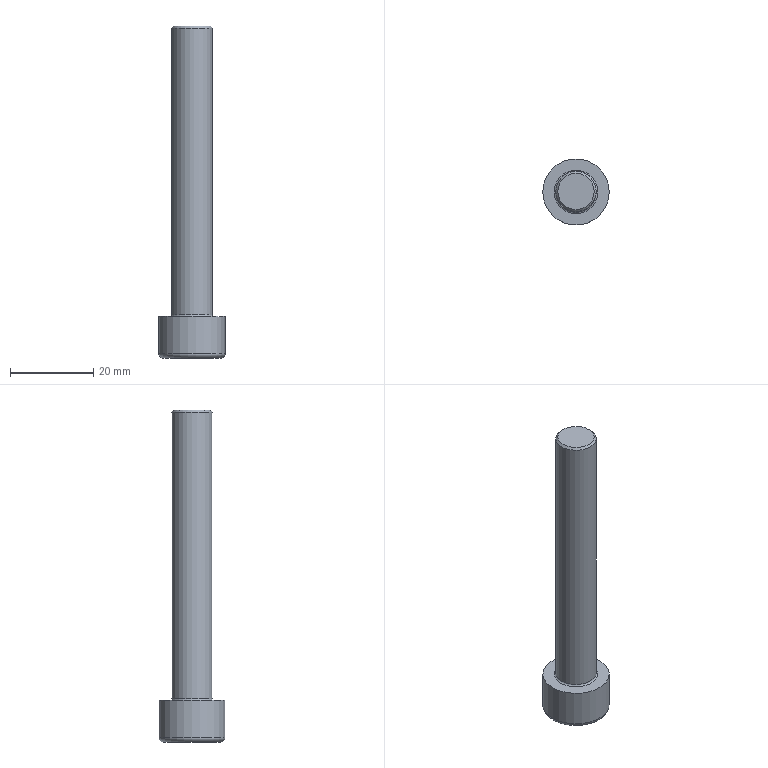Component | NX | GB-T70_1-2000_M10X70 | 1 solid | 27 faces | volume 6832 mm3 | plane 15 | cone 8 | cylinder 2 | torus 2 | commonest cylinder face diameters 9.732 x1 16 x1